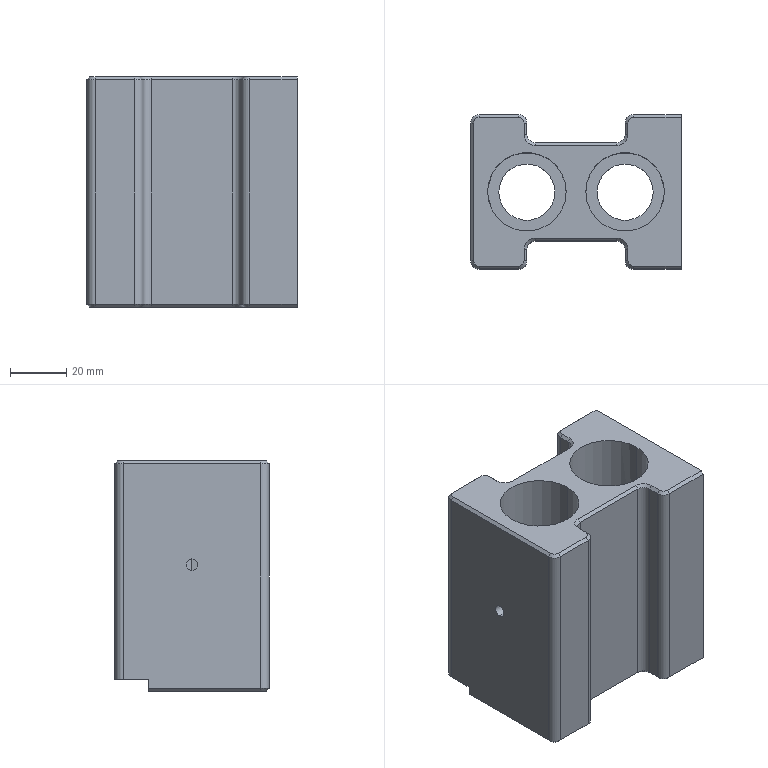Component | SolidWorks | DZ.KX.203-TC1505-30-09-01-05-01-2 | 1 solid | 102 faces | box 75 x 55 x 82 mm | volume 181065 mm3 | cylinder 38 | plane 37 | cone 27 | commonest cylinder face diameters 4.2 x16 6 x14 28 x4 20 x4
build123d program:
from build123d import *

# Parameters (mm, degrees)
SKETCH1_W                    = 82
SKETCH1_H                    = 55
BOSS_EXTRUDE1_DEPTH          = 75
M5_TAPPED_HOLE4_D            = 4.2
M5_TAPPED_HOLE4_DEPTH        = 17.4
M5_TAPPED_HOLE4_TIP          = 1.262
F_6_0_6_DIAMETER_HOLE1_D     = 6
F_6_0_6_DIAMETER_HOLE1_DEPTH = 10
HOLE1_D                      = 20
HOLE1_CBORE_D                = 28
HOLE1_CBORE_DEPTH            = 72
SKETCH21_W                   = 87.022
SKETCH21_H                   = 54.718
CUT_EXTRUDE1_DEPTH           = 4
M5_TAPPED_HOLE2_D            = 4.2
M5_TAPPED_HOLE2_DEPTH        = 10.4
M5_TAPPED_HOLE2_TIP          = 1.262
M5_TAPPED_HOLE3_D            = 4.2
M5_TAPPED_HOLE3_DEPTH        = 10.4
M5_TAPPED_HOLE3_TIP          = 1.262
SKETCH28_W                   = 35
SKETCH28_H                   = 10
CUT_EXTRUDE2_DEPTH           = 115.478
M5_TAPPED_HOLE5_D            = 4.2
M5_TAPPED_HOLE5_DEPTH        = 15
M5_TAPPED_HOLE5_TIP          = 1.262
FILLET1_R                    = 3
CHAMFER1_SIZE                = 1


with BuildPart() as part:
    # Sketch1 → Boss-Extrude1 (new body)
    with BuildSketch(Plane(origin=(0, 0, 0), x_dir=(0, 0, -1), z_dir=(1, 0, 0))):
        Rectangle(SKETCH1_W, SKETCH1_H)
    extrude(amount=BOSS_EXTRUDE1_DEPTH)

    # M5 Tapped Hole4
    with Locations(Plane(origin=(75, 0, 0), x_dir=(0, 0, 1), z_dir=(1, 0, 0))):
        with Locations((-28, 21), (-28, -21), (20, -21), (20, 21)):
            Hole(M5_TAPPED_HOLE4_D / 2, depth=M5_TAPPED_HOLE4_DEPTH)
            with Locations((0, 0, -(M5_TAPPED_HOLE4_DEPTH + M5_TAPPED_HOLE4_TIP / 2))):  # 118° drill point
                Cone(0, M5_TAPPED_HOLE4_D / 2, M5_TAPPED_HOLE4_TIP, mode=Mode.SUBTRACT)

    # 6.0 _6_ Diameter Hole1
    with Locations(Plane(origin=(75, 0, 0), x_dir=(0, 0, 1), z_dir=(1, 0, 0))):
        with Locations((-4, -21), (-4, 21)):
            Hole(F_6_0_6_DIAMETER_HOLE1_D / 2, depth=F_6_0_6_DIAMETER_HOLE1_DEPTH)

    # Hole1 (through all)
    with Locations(Plane(origin=(0, 0, -41), x_dir=(1, 0, 0), z_dir=(0, 0, -1))):
        with Locations((20, 0), (55, 0)):
            CounterBoreHole(HOLE1_D / 2, HOLE1_CBORE_D / 2, HOLE1_CBORE_DEPTH)

    # Sketch21 → Cut-Extrude1 (cut)
    with BuildSketch(Plane.XY.offset(41)):
        with Locations((35.97, -42.859)):
            Rectangle(SKETCH21_W, SKETCH21_H)
    extrude(amount=-CUT_EXTRUDE1_DEPTH, mode=Mode.SUBTRACT)

    # M5 Tapped Hole2
    with Locations(Plane(origin=(75, 0, 0), x_dir=(0, 0, -1), z_dir=(1, 0, 0))):
        with Locations((4, 0)):
            Hole(M5_TAPPED_HOLE2_D / 2, depth=M5_TAPPED_HOLE2_DEPTH)
            with Locations((0, 0, -(M5_TAPPED_HOLE2_DEPTH + M5_TAPPED_HOLE2_TIP / 2))):  # 118° drill point
                Cone(0, M5_TAPPED_HOLE2_D / 2, M5_TAPPED_HOLE2_TIP, mode=Mode.SUBTRACT)

    # M5 Tapped Hole3
    with Locations(Plane.ZY):
        with Locations((-4, 0)):
            Hole(M5_TAPPED_HOLE3_D / 2, depth=M5_TAPPED_HOLE3_DEPTH)
            with Locations((0, 0, -(M5_TAPPED_HOLE3_DEPTH + M5_TAPPED_HOLE3_TIP / 2))):  # 118° drill point
                Cone(0, M5_TAPPED_HOLE3_D / 2, M5_TAPPED_HOLE3_TIP, mode=Mode.SUBTRACT)

    # Sketch28 → Cut-Extrude2 (cut, through all)
    with BuildSketch(Plane(origin=(0, 0, -41), x_dir=(-1, 0, 0), z_dir=(0, 0, -1))):
        with Locations((-37.5, 22.5)):
            Rectangle(SKETCH28_W, SKETCH28_H)
        with Locations((-37.5, -22.5)):
            Rectangle(SKETCH28_W, SKETCH28_H)
    extrude(amount=-CUT_EXTRUDE2_DEPTH, mode=Mode.SUBTRACT)

    # M5 Tapped Hole5
    with Locations(Plane.XY.offset(37)):
        with Locations((12.5, -21.5), (62.5, -21.5)):
            Hole(M5_TAPPED_HOLE5_D / 2, depth=M5_TAPPED_HOLE5_DEPTH)
            with Locations((0, 0, -(M5_TAPPED_HOLE5_DEPTH + M5_TAPPED_HOLE5_TIP / 2))):  # 118° drill point
                Cone(0, M5_TAPPED_HOLE5_D / 2, M5_TAPPED_HOLE5_TIP, mode=Mode.SUBTRACT)

    # Fillet1
    fillet1_edges = [part.edges().sort_by_distance(p)[0] for p in [
        (20, -17.5, -2),
        (20, -27.5, -2),
        (55, -27.5, -2),
        (55, -17.5, -2),
        (0, 27.5, 0),
        (0, -27.5, -2),
        (55, 17.5, 0),
        (55, 27.5, 0),
        (20, 27.5, 0),
        (20, 17.5, 0),
    ]]
    fillet(fillet1_edges, radius=FILLET1_R)

    # Chamfer1
    chamfer1_edges = [part.edges().sort_by_distance(p)[0] for p in [
        (10, 27.5, 41),
        (10, 27.5, -41),
        (37.5, -17.5, -41),
        (20, -22.5, -41),
        (10, -27.5, -41),
        (0, 0, -41),
        (20, 22.5, -41),
        (37.5, 17.5, -41),
        (55, 22.5, -41),
        (55, -22.5, -41),
        (55.879, -26.621, -41),
        (55.879, 26.621, -41),
        (0.8787, -26.621, -41),
        (0.8787, 26.621, -41),
        (19.121, -26.621, -41),
        (19.121, 26.621, -41),
        (20, 22.5, 41),
        (55, 22.5, 41),
        (37.5, 17.5, 41),
        (0, 4.5, 41),
        (55.879, 26.621, 41),
        (0.8787, 26.621, 41),
        (19.121, 26.621, 41),
        (20.879, -18.379, -41),
        (20.879, 18.379, -41),
        (20.879, 18.379, 41),
        (54.121, 18.379, -41),
        (54.121, 18.379, 41),
        (54.121, -18.379, -41),
        (66.5, -27.5, -41),
        (66.5, 27.5, 41),
        (66.5, 27.5, -41),
    ]]
    chamfer(chamfer1_edges, length=CHAMFER1_SIZE)


solid = part.part

# Placed as in the assembly
solid = solid.moved(Location((257, -610.807, 90.441), (180, 0, 0)))